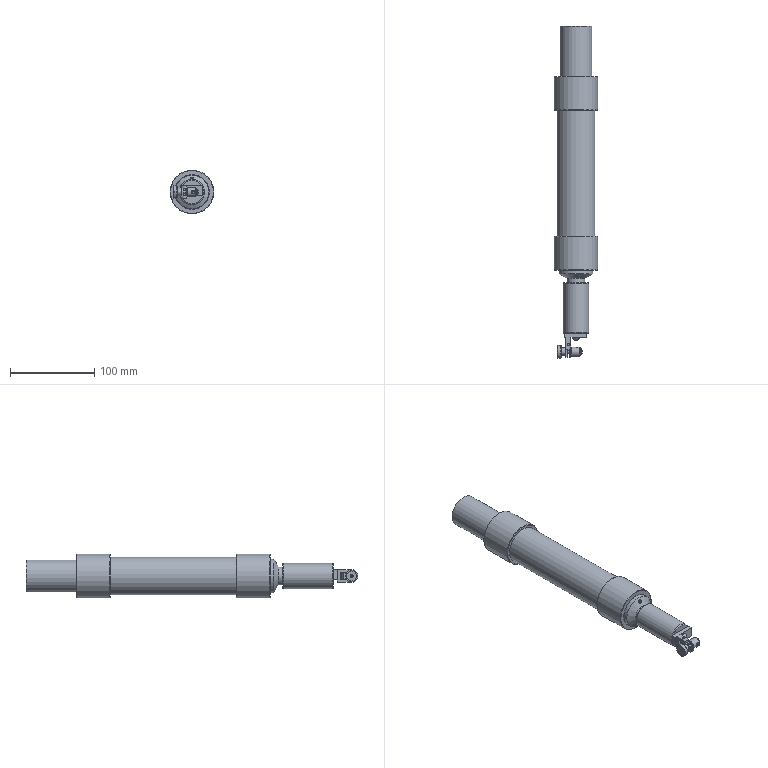Assembly | NX | mm | 17 component files | 17 solids | 183 faces | box 52 x 394.5 x 52 mm | volume 492069 mm3 | plane 74 | cylinder 57 | cone 27 | torus 20 | sphere 4 | spline 1 | commonest cylinder face diameters 4.2 x8 40 x6 8 x4 2.5 x4 3 x4 7 x3 10 x3 18 x2
Bill of materials:
GB99-86,5x16 | 1 |  | Slotted Round Head Wood Screw, GB 99-86,5x16
unnamed part 1 | 1 |  | Stepped cylindrical pin: a long slender shaft joined to a short, larger-diameter cylindrical head that has a transverse through hole and a domed end face.
unnamed part 2 | 1 |  | Thick-walled cylindrical sleeve with an axial through bore, chamfered outer ends and one transverse through hole across the body.
unnamed part 3 | 1 |  | Rectangular block with one rounded end, split lengthwise by a narrow slot that ends in a round relief hole, with a large transverse through hole crossing the two split jaws.
unnamed part 4 | 1 |  | Flanged bushing: a large-diameter disc flange with a smaller coaxial cylindrical boss and a small central through bore.
unnamed part 5 | 1 |  | Plain solid cylindrical rod with flat ends.
unnamed part 6 | 1 |  | Multi-diameter stepped shaft with a small pilot end, a conical transition, several cylindrical sections and small radial holes.
unnamed part 7 | 1 |  | Plain solid cylinder (short rod or slug) with flat ends.
unnamed part 8 | 1 |  | Solid cylinder with a small central axial hole and slightly rounded or chamfered end edges.
unnamed part 9 | 1 |  | Solid cylindrical pin with chamfered ends and a small rectangular notch or step cut into one end edge.
unnamed part 10 | 2 |  | Solid cylindrical pin with a rectangular slot cut across one end, a slight diameter step near that end, and small chamfers.
unnamed part 11 | 2 |  | Thin-walled plain cylindrical tube or sleeve with a uniform bore.
unnamed part 12 | 1 |  | Prismatic bracket: a rectangular plate with one round through hole, joined at right angles to a web carrying two parallel fork lugs with rounded ends and coaxial small holes.
unnamed part 13 | 2 |  | Solid sphere with a plain, featureless surface; rendered as a faceted tessellated mesh.
Mates:
1. concentric | 8_sleeve 1 edge | 9_mandrel 1 edge
2. concentric | 15_gauge_holder 1 edge | 8_sleeve 1 arc
3. fix | 9_mandrel 1 component
4. concentric | 3_gauge_base 1 edge | 15_gauge_holder 1 edge
5. touch align | 4_gauge_clamp_pin 1 face | 5_gauge_clamp_sleeve 1 face
6. touch align | 4_gauge_clamp_pin 1 face | 5_gauge_clamp_sleeve 1 face
7. touch align | 4_gauge_clamp_pin 1 face | 3_gauge_base 1 face
8. touch align | 5_gauge_clamp_sleeve 1 face | 3_gauge_base 1 face
9. concentric | 2_knurled_nut 1 arc | 3_gauge_base 1 edge
10. concentric | 1_small_shaft 1 edge | 15_gauge_holder 1 edge
11. concentric | 7_half_round_screw_M5x15 1 edge | 15_gauge_holder 1 edge
12. concentric | 10_thin_sleeve 2 edge | 9_mandrel 1 edge
13. concentric | 10_thin_sleeve 1 edge | 9_mandrel 1 edge
14. concentric | 12_pressure_pin 1 edge | 9_mandrel 1 edge
15. touch align | 13_steel_ball 2 face | 9_mandrel 1 face
16. touch align | 13_steel_ball 2 face | 9_mandrel 1 edge
17. touch align | 13_steel_ball 1 face | 9_mandrel 1 face
18. touch align | 13_steel_ball 1 face | 9_mandrel 1 edge
19. concentric | 14_air_plug 1 edge | 9_mandrel 1 edge
20. touch align | 14_air_plug 2 face | 9_mandrel 1 face
21. concentric | 11_small_piston 1 edge | 9_mandrel 1 edge